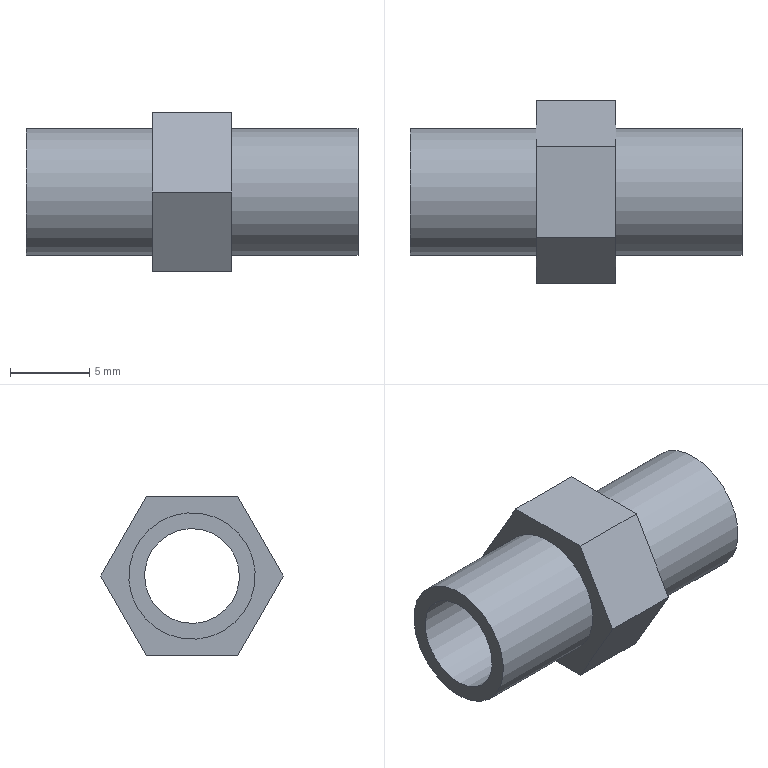Component | NX | PIPE_CAP_INTERFACE | 1 solid | 13 faces | box 21 x 11.55 x 10 mm | volume 643 mm3 | plane 10 | cylinder 3 | commonest cylinder face diameters 8 x2 6 x1
STEP:
#1=CARTESIAN_POINT('',(0.,0.,0.));
#2=DIRECTION('',(0.,0.,1.));
#3=DIRECTION('',(1.,0.,0.));
#4=AXIS2_PLACEMENT_3D('',#1,#2,#3);
#5=CARTESIAN_POINT('',(104.,-9.25,43.598));
#6=VERTEX_POINT('',#5);
#7=CARTESIAN_POINT('',(104.,-12.25,38.402));
#8=VERTEX_POINT('',#7);
#9=CARTESIAN_POINT('',(104.,-10.75,41.));
#10=DIRECTION('',(-1.,0.,0.));
#11=DIRECTION('',(0.,0.5,0.866));
#12=AXIS2_PLACEMENT_3D('',#9,#10,#11);
#13=CIRCLE('',#12,3.);
#14=CARTESIAN_POINT('',(104.,-10.75,41.));
#15=DIRECTION('',(-1.,0.,0.));
#16=DIRECTION('',(0.,0.5,0.866));
#17=AXIS2_PLACEMENT_3D('',#14,#15,#16);
#18=PLANE('',#17);
#19=CARTESIAN_POINT('',(0.,0.));
#20=DIRECTION('',(1.,0.));
#21=AXIS2_PLACEMENT_2D('',#19,#20);
#22=CIRCLE('',#21,3.);
#23=(GEOMETRIC_REPRESENTATION_CONTEXT(2)PARAMETRIC_REPRESENTATION_CONTEXT()REPRESENTATION_CONTEXT('',''));
#24=DEFINITIONAL_REPRESENTATION('',(#22),#23);
#25=PCURVE('',#18,#24);
#26=CARTESIAN_POINT('',(100.5,-10.75,41.));
#27=DIRECTION('',(1.,0.,0.));
#28=DIRECTION('',(0.,-0.5,-0.866));
#29=AXIS2_PLACEMENT_3D('',#26,#27,#28);
#30=CYLINDRICAL_SURFACE('',#29,3.);
#31=CARTESIAN_POINT('',(3.142,3.5));
#32=DIRECTION('',(-1.,0.));
#33=VECTOR('',#32,1.);
#34=LINE('',#31,#33);
#35=(GEOMETRIC_REPRESENTATION_CONTEXT(2)PARAMETRIC_REPRESENTATION_CONTEXT()REPRESENTATION_CONTEXT('',''));
#36=DEFINITIONAL_REPRESENTATION('',(#34),#35);
#37=PCURVE('',#30,#36);
#38=SURFACE_CURVE('',#13,(#25,#37),.PCURVE_S1.);
#39=EDGE_CURVE('',#6,#8,#38,.T.);
#40=ORIENTED_EDGE('',*,*,#39,.F.);
#41=CARTESIAN_POINT('',(104.,-10.75,41.));
#42=DIRECTION('',(-1.,0.,0.));
#43=DIRECTION('',(0.,0.5,0.866));
#44=AXIS2_PLACEMENT_3D('',#41,#42,#43);
#45=CIRCLE('',#44,3.);
#46=CARTESIAN_POINT('',(0.,0.));
#47=DIRECTION('',(1.,0.));
#48=AXIS2_PLACEMENT_2D('',#46,#47);
#49=CIRCLE('',#48,3.);
#50=(GEOMETRIC_REPRESENTATION_CONTEXT(2)PARAMETRIC_REPRESENTATION_CONTEXT()REPRESENTATION_CONTEXT('',''));
#51=DEFINITIONAL_REPRESENTATION('',(#49),#50);
#52=PCURVE('',#18,#51);
#53=CARTESIAN_POINT('',(9.425,3.5));
#54=DIRECTION('',(-1.,0.));
#55=VECTOR('',#54,1.);
#56=LINE('',#53,#55);
#57=(GEOMETRIC_REPRESENTATION_CONTEXT(2)PARAMETRIC_REPRESENTATION_CONTEXT()REPRESENTATION_CONTEXT('',''));
#58=DEFINITIONAL_REPRESENTATION('',(#56),#57);
#59=PCURVE('',#30,#58);
#60=SURFACE_CURVE('',#45,(#52,#59),.PCURVE_S1.);
#61=EDGE_CURVE('',#8,#6,#60,.T.);
#62=ORIENTED_EDGE('',*,*,#61,.F.);
#63=EDGE_LOOP('',(#40,#62));
#64=FACE_BOUND('',#63,.T.);
#65=CARTESIAN_POINT('',(104.,-12.75,37.536));
#66=VERTEX_POINT('',#65);
#67=CARTESIAN_POINT('',(104.,-10.75,41.));
#68=DIRECTION('',(1.,0.,0.));
#69=DIRECTION('',(0.,-0.5,-0.866));
#70=AXIS2_PLACEMENT_3D('',#67,#68,#69);
#71=CIRCLE('',#70,4.);
#72=CARTESIAN_POINT('',(-4.,0.));
#73=CARTESIAN_POINT('',(-4.,6.928));
#74=CARTESIAN_POINT('',(2.,3.464));
#75=CARTESIAN_POINT('',(8.,0.));
#76=CARTESIAN_POINT('',(2.,-3.464));
#77=CARTESIAN_POINT('',(-4.,-6.928));
#78=CARTESIAN_POINT('',(-4.,0.));
#79=(BOUNDED_CURVE()B_SPLINE_CURVE(2,(#72,#73,#74,#75,#76,#77,#78),.UNSPECIFIED.,.T.,.F.)B_SPLINE_CURVE_WITH_KNOTS((1,2,2,2,2,1),(-2.094,0.,2.094,4.189,6.283,8.378),.UNSPECIFIED.)CURVE()GEOMETRIC_REPRESENTATION_ITEM()RATIONAL_B_SPLINE_CURVE((1.,0.5,1.,0.5,1.,0.5,1.))REPRESENTATION_ITEM(''));
#80=(GEOMETRIC_REPRESENTATION_CONTEXT(2)PARAMETRIC_REPRESENTATION_CONTEXT()REPRESENTATION_CONTEXT('',''));
#81=DEFINITIONAL_REPRESENTATION('',(#79),#80);
#82=PCURVE('',#18,#81);
#83=CARTESIAN_POINT('',(104.,-10.75,41.));
#84=DIRECTION('',(1.,0.,0.));
#85=DIRECTION('',(0.,-0.5,-0.866));
#86=AXIS2_PLACEMENT_3D('',#83,#84,#85);
#87=CYLINDRICAL_SURFACE('',#86,4.);
#88=CARTESIAN_POINT('',(0.,0.));
#89=DIRECTION('',(1.,0.));
#90=VECTOR('',#89,1.);
#91=LINE('',#88,#90);
#92=(GEOMETRIC_REPRESENTATION_CONTEXT(2)PARAMETRIC_REPRESENTATION_CONTEXT()REPRESENTATION_CONTEXT('',''));
#93=DEFINITIONAL_REPRESENTATION('',(#91),#92);
#94=PCURVE('',#87,#93);
#95=SURFACE_CURVE('',#71,(#82,#94),.PCURVE_S1.);
#96=EDGE_CURVE('',#66,#66,#95,.T.);
#97=ORIENTED_EDGE('',*,*,#96,.F.);
#98=EDGE_LOOP('',(#97));
#99=FACE_BOUND('',#98,.T.);
#100=ADVANCED_FACE('',(#64,#99),#18,.T.);
#101=CARTESIAN_POINT('',(112.,-12.75,37.536));
#102=VERTEX_POINT('',#101);
#103=CARTESIAN_POINT('',(112.,-10.75,41.));
#104=DIRECTION('',(-1.,0.,0.));
#105=DIRECTION('',(0.,-0.5,-0.866));
#106=AXIS2_PLACEMENT_3D('',#103,#104,#105);
#107=CIRCLE('',#106,4.);
#108=CARTESIAN_POINT('',(6.283,8.));
#109=DIRECTION('',(-1.,0.));
#110=VECTOR('',#109,1.);
#111=LINE('',#108,#110);
#112=(GEOMETRIC_REPRESENTATION_CONTEXT(2)PARAMETRIC_REPRESENTATION_CONTEXT()REPRESENTATION_CONTEXT('',''));
#113=DEFINITIONAL_REPRESENTATION('',(#111),#112);
#114=PCURVE('',#87,#113);
#115=CARTESIAN_POINT('',(112.,-10.75,41.));
#116=DIRECTION('',(1.,0.,0.));
#117=DIRECTION('',(0.,-0.5,-0.866));
#118=AXIS2_PLACEMENT_3D('',#115,#116,#117);
#119=PLANE('',#118);
#120=CARTESIAN_POINT('',(4.,0.));
#121=CARTESIAN_POINT('',(4.,-6.928));
#122=CARTESIAN_POINT('',(-2.,-3.464));
#123=CARTESIAN_POINT('',(-8.,-0.));
#124=CARTESIAN_POINT('',(-2.,3.464));
#125=CARTESIAN_POINT('',(4.,6.928));
#126=CARTESIAN_POINT('',(4.,0.));
#127=(BOUNDED_CURVE()B_SPLINE_CURVE(2,(#120,#121,#122,#123,#124,#125,#126),.UNSPECIFIED.,.T.,.F.)B_SPLINE_CURVE_WITH_KNOTS((1,2,2,2,2,1),(-2.094,0.,2.094,4.189,6.283,8.378),.UNSPECIFIED.)CURVE()GEOMETRIC_REPRESENTATION_ITEM()RATIONAL_B_SPLINE_CURVE((1.,0.5,1.,0.5,1.,0.5,1.))REPRESENTATION_ITEM(''));
#128=(GEOMETRIC_REPRESENTATION_CONTEXT(2)PARAMETRIC_REPRESENTATION_CONTEXT()REPRESENTATION_CONTEXT('',''));
#129=DEFINITIONAL_REPRESENTATION('',(#127),#128);
#130=PCURVE('',#119,#129);
#131=SURFACE_CURVE('',#107,(#114,#130),.PCURVE_S1.);
#132=EDGE_CURVE('',#102,#102,#131,.T.);
#133=ORIENTED_EDGE('',*,*,#132,.T.);
#134=CARTESIAN_POINT('',(104.,-12.75,37.536));
#135=CARTESIAN_POINT('',(112.,-12.75,37.536));
#136=B_SPLINE_CURVE_WITH_KNOTS('',1,(#134,#135),.UNSPECIFIED.,.F.,.F.,(2,2),(0.,8.),.PIECEWISE_BEZIER_KNOTS.);
#137=CARTESIAN_POINT('',(0.,0.));
#138=DIRECTION('',(0.,1.));
#139=VECTOR('',#138,1.);
#140=LINE('',#137,#139);
#141=(GEOMETRIC_REPRESENTATION_CONTEXT(2)PARAMETRIC_REPRESENTATION_CONTEXT()REPRESENTATION_CONTEXT('',''));
#142=DEFINITIONAL_REPRESENTATION('',(#140),#141);
#143=PCURVE('',#87,#142);
#144=CARTESIAN_POINT('',(6.283,0.));
#145=DIRECTION('',(0.,1.));
#146=VECTOR('',#145,1.);
#147=LINE('',#144,#146);
#148=(GEOMETRIC_REPRESENTATION_CONTEXT(2)PARAMETRIC_REPRESENTATION_CONTEXT()REPRESENTATION_CONTEXT('',''));
#149=DEFINITIONAL_REPRESENTATION('',(#147),#148);
#150=PCURVE('',#87,#149);
#151=SEAM_CURVE('',#136,(#143,#150),.PCURVE_S1.);
#152=EDGE_CURVE('',#66,#102,#151,.T.);
#153=ORIENTED_EDGE('',*,*,#152,.F.);
#154=ORIENTED_EDGE('',*,*,#96,.T.);
#155=ORIENTED_EDGE('',*,*,#152,.T.);
#156=EDGE_LOOP('',(#133,#153,#154,#155));
#157=FACE_BOUND('',#156,.T.);
#158=ADVANCED_FACE('',(#157),#87,.T.);
#159=CARTESIAN_POINT('',(112.,-7.863,36.));
#160=VERTEX_POINT('',#159);
#161=CARTESIAN_POINT('',(112.,-4.976,41.));
#162=VERTEX_POINT('',#161);
#163=CARTESIAN_POINT('',(112.,-7.863,36.));
#164=DIRECTION('',(0.,0.5,0.866));
#165=VECTOR('',#164,1.);
#166=LINE('',#163,#165);
#167=CARTESIAN_POINT('',(117.,-7.863,36.));
#168=DIRECTION('',(0.,-0.866,0.5));
#169=DIRECTION('',(0.,-0.5,-0.866));
#170=AXIS2_PLACEMENT_3D('',#167,#168,#169);
#171=PLANE('',#170);
#172=CARTESIAN_POINT('',(0.,-5.));
#173=DIRECTION('',(-1.,0.));
#174=VECTOR('',#173,1.);
#175=LINE('',#172,#174);
#176=(GEOMETRIC_REPRESENTATION_CONTEXT(2)PARAMETRIC_REPRESENTATION_CONTEXT()REPRESENTATION_CONTEXT('',''));
#177=DEFINITIONAL_REPRESENTATION('',(#175),#176);
#178=PCURVE('',#171,#177);
#179=CARTESIAN_POINT('',(2.887,5.));
#180=DIRECTION('',(-1.,0.));
#181=VECTOR('',#180,1.);
#182=LINE('',#179,#181);
#183=(GEOMETRIC_REPRESENTATION_CONTEXT(2)PARAMETRIC_REPRESENTATION_CONTEXT()REPRESENTATION_CONTEXT('',''));
#184=DEFINITIONAL_REPRESENTATION('',(#182),#183);
#185=PCURVE('',#119,#184);
#186=SURFACE_CURVE('',#166,(#178,#185),.PCURVE_S1.);
#187=EDGE_CURVE('',#160,#162,#186,.T.);
#188=ORIENTED_EDGE('',*,*,#187,.T.);
#189=CARTESIAN_POINT('',(117.,-4.976,41.));
#190=VERTEX_POINT('',#189);
#191=CARTESIAN_POINT('',(117.,-4.976,41.));
#192=DIRECTION('',(-1.,0.,0.));
#193=VECTOR('',#192,1.);
#194=LINE('',#191,#193);
#195=CARTESIAN_POINT('',(-5.774,0.));
#196=DIRECTION('',(0.,-1.));
#197=VECTOR('',#196,1.);
#198=LINE('',#195,#197);
#199=(GEOMETRIC_REPRESENTATION_CONTEXT(2)PARAMETRIC_REPRESENTATION_CONTEXT()REPRESENTATION_CONTEXT('',''));
#200=DEFINITIONAL_REPRESENTATION('',(#198),#199);
#201=PCURVE('',#171,#200);
#202=CARTESIAN_POINT('',(117.,-4.976,41.));
#203=DIRECTION('',(0.,-0.866,-0.5));
#204=DIRECTION('',(0.,0.5,-0.866));
#205=AXIS2_PLACEMENT_3D('',#202,#203,#204);
#206=PLANE('',#205);
#207=CARTESIAN_POINT('',(0.,0.));
#208=DIRECTION('',(0.,-1.));
#209=VECTOR('',#208,1.);
#210=LINE('',#207,#209);
#211=(GEOMETRIC_REPRESENTATION_CONTEXT(2)PARAMETRIC_REPRESENTATION_CONTEXT()REPRESENTATION_CONTEXT('',''));
#212=DEFINITIONAL_REPRESENTATION('',(#210),#211);
#213=PCURVE('',#206,#212);
#214=SURFACE_CURVE('',#194,(#201,#213),.PCURVE_S1.);
#215=EDGE_CURVE('',#190,#162,#214,.T.);
#216=ORIENTED_EDGE('',*,*,#215,.F.);
#217=CARTESIAN_POINT('',(117.,-7.863,36.));
#218=VERTEX_POINT('',#217);
#219=CARTESIAN_POINT('',(117.,-7.863,36.));
#220=DIRECTION('',(0.,0.5,0.866));
#221=VECTOR('',#220,1.);
#222=LINE('',#219,#221);
#223=CARTESIAN_POINT('',(0.,0.));
#224=DIRECTION('',(-1.,0.));
#225=VECTOR('',#224,1.);
#226=LINE('',#223,#225);
#227=(GEOMETRIC_REPRESENTATION_CONTEXT(2)PARAMETRIC_REPRESENTATION_CONTEXT()REPRESENTATION_CONTEXT('',''));
#228=DEFINITIONAL_REPRESENTATION('',(#226),#227);
#229=PCURVE('',#171,#228);
#230=CARTESIAN_POINT('',(117.,-10.75,41.));
#231=DIRECTION('',(1.,0.,0.));
#232=DIRECTION('',(0.,-0.5,-0.866));
#233=AXIS2_PLACEMENT_3D('',#230,#231,#232);
#234=PLANE('',#233);
#235=CARTESIAN_POINT('',(2.887,5.));
#236=DIRECTION('',(-1.,0.));
#237=VECTOR('',#236,1.);
#238=LINE('',#235,#237);
#239=(GEOMETRIC_REPRESENTATION_CONTEXT(2)PARAMETRIC_REPRESENTATION_CONTEXT()REPRESENTATION_CONTEXT('',''));
#240=DEFINITIONAL_REPRESENTATION('',(#238),#239);
#241=PCURVE('',#234,#240);
#242=SURFACE_CURVE('',#222,(#229,#241),.PCURVE_S1.);
#243=EDGE_CURVE('',#218,#190,#242,.T.);
#244=ORIENTED_EDGE('',*,*,#243,.F.);
#245=CARTESIAN_POINT('',(117.,-7.863,36.));
#246=DIRECTION('',(-1.,0.,0.));
#247=VECTOR('',#246,1.);
#248=LINE('',#245,#247);
#249=CARTESIAN_POINT('',(0.,0.));
#250=DIRECTION('',(0.,-1.));
#251=VECTOR('',#250,1.);
#252=LINE('',#249,#251);
#253=(GEOMETRIC_REPRESENTATION_CONTEXT(2)PARAMETRIC_REPRESENTATION_CONTEXT()REPRESENTATION_CONTEXT('',''));
#254=DEFINITIONAL_REPRESENTATION('',(#252),#253);
#255=PCURVE('',#171,#254);
#256=CARTESIAN_POINT('',(117.,-13.637,36.));
#257=DIRECTION('',(0.,0.,1.));
#258=DIRECTION('',(0.,-1.,0.));
#259=AXIS2_PLACEMENT_3D('',#256,#257,#258);
#260=PLANE('',#259);
#261=CARTESIAN_POINT('',(-5.774,0.));
#262=DIRECTION('',(0.,-1.));
#263=VECTOR('',#262,1.);
#264=LINE('',#261,#263);
#265=(GEOMETRIC_REPRESENTATION_CONTEXT(2)PARAMETRIC_REPRESENTATION_CONTEXT()REPRESENTATION_CONTEXT('',''));
#266=DEFINITIONAL_REPRESENTATION('',(#264),#265);
#267=PCURVE('',#260,#266);
#268=SURFACE_CURVE('',#248,(#255,#267),.PCURVE_S1.);
#269=EDGE_CURVE('',#218,#160,#268,.T.);
#270=ORIENTED_EDGE('',*,*,#269,.T.);
#271=EDGE_LOOP('',(#188,#216,#244,#270));
#272=FACE_BOUND('',#271,.T.);
#273=ADVANCED_FACE('',(#272),#171,.F.);
#274=CARTESIAN_POINT('',(112.,-7.863,46.));
#275=VERTEX_POINT('',#274);
#276=CARTESIAN_POINT('',(112.,-4.976,41.));
#277=DIRECTION('',(0.,-0.5,0.866));
#278=VECTOR('',#277,1.);
#279=LINE('',#276,#278);
#280=CARTESIAN_POINT('',(0.,-5.));
#281=DIRECTION('',(-1.,0.));
#282=VECTOR('',#281,1.);
#283=LINE('',#280,#282);
#284=(GEOMETRIC_REPRESENTATION_CONTEXT(2)PARAMETRIC_REPRESENTATION_CONTEXT()REPRESENTATION_CONTEXT('',''));
#285=DEFINITIONAL_REPRESENTATION('',(#283),#284);
#286=PCURVE('',#206,#285);
#287=CARTESIAN_POINT('',(-2.887,5.));
#288=DIRECTION('',(-0.5,-0.866));
#289=VECTOR('',#288,1.);
#290=LINE('',#287,#289);
#291=(GEOMETRIC_REPRESENTATION_CONTEXT(2)PARAMETRIC_REPRESENTATION_CONTEXT()REPRESENTATION_CONTEXT('',''));
#292=DEFINITIONAL_REPRESENTATION('',(#290),#291);
#293=PCURVE('',#119,#292);
#294=SURFACE_CURVE('',#279,(#286,#293),.PCURVE_S1.);
#295=EDGE_CURVE('',#162,#275,#294,.T.);
#296=ORIENTED_EDGE('',*,*,#295,.T.);
#297=CARTESIAN_POINT('',(117.,-7.863,46.));
#298=VERTEX_POINT('',#297);
#299=CARTESIAN_POINT('',(117.,-7.863,46.));
#300=DIRECTION('',(-1.,0.,0.));
#301=VECTOR('',#300,1.);
#302=LINE('',#299,#301);
#303=CARTESIAN_POINT('',(-5.774,0.));
#304=DIRECTION('',(0.,-1.));
#305=VECTOR('',#304,1.);
#306=LINE('',#303,#305);
#307=(GEOMETRIC_REPRESENTATION_CONTEXT(2)PARAMETRIC_REPRESENTATION_CONTEXT()REPRESENTATION_CONTEXT('',''));
#308=DEFINITIONAL_REPRESENTATION('',(#306),#307);
#309=PCURVE('',#206,#308);
#310=CARTESIAN_POINT('',(117.,-7.863,46.));
#311=DIRECTION('',(0.,-0.,-1.));
#312=DIRECTION('',(0.,1.,-0.));
#313=AXIS2_PLACEMENT_3D('',#310,#311,#312);
#314=PLANE('',#313);
#315=CARTESIAN_POINT('',(0.,0.));
#316=DIRECTION('',(0.,-1.));
#317=VECTOR('',#316,1.);
#318=LINE('',#315,#317);
#319=(GEOMETRIC_REPRESENTATION_CONTEXT(2)PARAMETRIC_REPRESENTATION_CONTEXT()REPRESENTATION_CONTEXT('',''));
#320=DEFINITIONAL_REPRESENTATION('',(#318),#319);
#321=PCURVE('',#314,#320);
#322=SURFACE_CURVE('',#302,(#309,#321),.PCURVE_S1.);
#323=EDGE_CURVE('',#298,#275,#322,.T.);
#324=ORIENTED_EDGE('',*,*,#323,.F.);
#325=CARTESIAN_POINT('',(117.,-4.976,41.));
#326=DIRECTION('',(0.,-0.5,0.866));
#327=VECTOR('',#326,1.);
#328=LINE('',#325,#327);
#329=CARTESIAN_POINT('',(0.,0.));
#330=DIRECTION('',(-1.,0.));
#331=VECTOR('',#330,1.);
#332=LINE('',#329,#331);
#333=(GEOMETRIC_REPRESENTATION_CONTEXT(2)PARAMETRIC_REPRESENTATION_CONTEXT()REPRESENTATION_CONTEXT('',''));
#334=DEFINITIONAL_REPRESENTATION('',(#332),#333);
#335=PCURVE('',#206,#334);
#336=CARTESIAN_POINT('',(-2.887,5.));
#337=DIRECTION('',(-0.5,-0.866));
#338=VECTOR('',#337,1.);
#339=LINE('',#336,#338);
#340=(GEOMETRIC_REPRESENTATION_CONTEXT(2)PARAMETRIC_REPRESENTATION_CONTEXT()REPRESENTATION_CONTEXT('',''));
#341=DEFINITIONAL_REPRESENTATION('',(#339),#340);
#342=PCURVE('',#234,#341);
#343=SURFACE_CURVE('',#328,(#335,#342),.PCURVE_S1.);
#344=EDGE_CURVE('',#190,#298,#343,.T.);
#345=ORIENTED_EDGE('',*,*,#344,.F.);
#346=ORIENTED_EDGE('',*,*,#215,.T.);
#347=EDGE_LOOP('',(#296,#324,#345,#346));
#348=FACE_BOUND('',#347,.T.);
#349=ADVANCED_FACE('',(#348),#206,.F.);
#350=CARTESIAN_POINT('',(112.,-13.637,46.));
#351=VERTEX_POINT('',#350);
#352=CARTESIAN_POINT('',(112.,-7.863,46.));
#353=DIRECTION('',(0.,-1.,0.));
#354=VECTOR('',#353,1.);
#355=LINE('',#352,#354);
#356=CARTESIAN_POINT('',(0.,-5.));
#357=DIRECTION('',(-1.,0.));
#358=VECTOR('',#357,1.);
#359=LINE('',#356,#358);
#360=(GEOMETRIC_REPRESENTATION_CONTEXT(2)PARAMETRIC_REPRESENTATION_CONTEXT()REPRESENTATION_CONTEXT('',''));
#361=DEFINITIONAL_REPRESENTATION('',(#359),#360);
#362=PCURVE('',#314,#361);
#363=CARTESIAN_POINT('',(-5.774,-0.));
#364=DIRECTION('',(0.5,-0.866));
#365=VECTOR('',#364,1.);
#366=LINE('',#363,#365);
#367=(GEOMETRIC_REPRESENTATION_CONTEXT(2)PARAMETRIC_REPRESENTATION_CONTEXT()REPRESENTATION_CONTEXT('',''));
#368=DEFINITIONAL_REPRESENTATION('',(#366),#367);
#369=PCURVE('',#119,#368);
#370=SURFACE_CURVE('',#355,(#362,#369),.PCURVE_S1.);
#371=EDGE_CURVE('',#275,#351,#370,.T.);
#372=ORIENTED_EDGE('',*,*,#371,.T.);
#373=CARTESIAN_POINT('',(117.,-13.637,46.));
#374=VERTEX_POINT('',#373);
#375=CARTESIAN_POINT('',(117.,-13.637,46.));
#376=DIRECTION('',(-1.,0.,0.));
#377=VECTOR('',#376,1.);
#378=LINE('',#375,#377);
#379=CARTESIAN_POINT('',(-5.774,0.));
#380=DIRECTION('',(0.,-1.));
#381=VECTOR('',#380,1.);
#382=LINE('',#379,#381);
#383=(GEOMETRIC_REPRESENTATION_CONTEXT(2)PARAMETRIC_REPRESENTATION_CONTEXT()REPRESENTATION_CONTEXT('',''));
#384=DEFINITIONAL_REPRESENTATION('',(#382),#383);
#385=PCURVE('',#314,#384);
#386=CARTESIAN_POINT('',(117.,-13.637,46.));
#387=DIRECTION('',(0.,0.866,-0.5));
#388=DIRECTION('',(0.,0.5,0.866));
#389=AXIS2_PLACEMENT_3D('',#386,#387,#388);
#390=PLANE('',#389);
#391=CARTESIAN_POINT('',(0.,0.));
#392=DIRECTION('',(0.,-1.));
#393=VECTOR('',#392,1.);
#394=LINE('',#391,#393);
#395=(GEOMETRIC_REPRESENTATION_CONTEXT(2)PARAMETRIC_REPRESENTATION_CONTEXT()REPRESENTATION_CONTEXT('',''));
#396=DEFINITIONAL_REPRESENTATION('',(#394),#395);
#397=PCURVE('',#390,#396);
#398=SURFACE_CURVE('',#378,(#385,#397),.PCURVE_S1.);
#399=EDGE_CURVE('',#374,#351,#398,.T.);
#400=ORIENTED_EDGE('',*,*,#399,.F.);
#401=CARTESIAN_POINT('',(117.,-7.863,46.));
#402=DIRECTION('',(0.,-1.,0.));
#403=VECTOR('',#402,1.);
#404=LINE('',#401,#403);
#405=CARTESIAN_POINT('',(0.,0.));
#406=DIRECTION('',(-1.,0.));
#407=VECTOR('',#406,1.);
#408=LINE('',#405,#407);
#409=(GEOMETRIC_REPRESENTATION_CONTEXT(2)PARAMETRIC_REPRESENTATION_CONTEXT()REPRESENTATION_CONTEXT('',''));
#410=DEFINITIONAL_REPRESENTATION('',(#408),#409);
#411=PCURVE('',#314,#410);
#412=CARTESIAN_POINT('',(-5.774,-0.));
#413=DIRECTION('',(0.5,-0.866));
#414=VECTOR('',#413,1.);
#415=LINE('',#412,#414);
#416=(GEOMETRIC_REPRESENTATION_CONTEXT(2)PARAMETRIC_REPRESENTATION_CONTEXT()REPRESENTATION_CONTEXT('',''));
#417=DEFINITIONAL_REPRESENTATION('',(#415),#416);
#418=PCURVE('',#234,#417);
#419=SURFACE_CURVE('',#404,(#411,#418),.PCURVE_S1.);
#420=EDGE_CURVE('',#298,#374,#419,.T.);
#421=ORIENTED_EDGE('',*,*,#420,.F.);
#422=ORIENTED_EDGE('',*,*,#323,.T.);
#423=EDGE_LOOP('',(#372,#400,#421,#422));
#424=FACE_BOUND('',#423,.T.);
#425=ADVANCED_FACE('',(#424),#314,.F.);
#426=CARTESIAN_POINT('',(112.,-16.524,41.));
#427=VERTEX_POINT('',#426);
#428=CARTESIAN_POINT('',(112.,-13.637,46.));
#429=DIRECTION('',(0.,-0.5,-0.866));
#430=VECTOR('',#429,1.);
#431=LINE('',#428,#430);
#432=CARTESIAN_POINT('',(0.,-5.));
#433=DIRECTION('',(-1.,0.));
#434=VECTOR('',#433,1.);
#435=LINE('',#432,#434);
#436=(GEOMETRIC_REPRESENTATION_CONTEXT(2)PARAMETRIC_REPRESENTATION_CONTEXT()REPRESENTATION_CONTEXT('',''));
#437=DEFINITIONAL_REPRESENTATION('',(#435),#436);
#438=PCURVE('',#390,#437);
#439=CARTESIAN_POINT('',(-2.887,-5.));
#440=DIRECTION('',(1.,-0.));
#441=VECTOR('',#440,1.);
#442=LINE('',#439,#441);
#443=(GEOMETRIC_REPRESENTATION_CONTEXT(2)PARAMETRIC_REPRESENTATION_CONTEXT()REPRESENTATION_CONTEXT('',''));
#444=DEFINITIONAL_REPRESENTATION('',(#442),#443);
#445=PCURVE('',#119,#444);
#446=SURFACE_CURVE('',#431,(#438,#445),.PCURVE_S1.);
#447=EDGE_CURVE('',#351,#427,#446,.T.);
#448=ORIENTED_EDGE('',*,*,#447,.T.);
#449=CARTESIAN_POINT('',(117.,-16.524,41.));
#450=VERTEX_POINT('',#449);
#451=CARTESIAN_POINT('',(117.,-16.524,41.));
#452=DIRECTION('',(-1.,0.,0.));
#453=VECTOR('',#452,1.);
#454=LINE('',#451,#453);
#455=CARTESIAN_POINT('',(-5.774,0.));
#456=DIRECTION('',(0.,-1.));
#457=VECTOR('',#456,1.);
#458=LINE('',#455,#457);
#459=(GEOMETRIC_REPRESENTATION_CONTEXT(2)PARAMETRIC_REPRESENTATION_CONTEXT()REPRESENTATION_CONTEXT('',''));
#460=DEFINITIONAL_REPRESENTATION('',(#458),#459);
#461=PCURVE('',#390,#460);
#462=CARTESIAN_POINT('',(117.,-16.524,41.));
#463=DIRECTION('',(0.,0.866,0.5));
#464=DIRECTION('',(0.,-0.5,0.866));
#465=AXIS2_PLACEMENT_3D('',#462,#463,#464);
#466=PLANE('',#465);
#467=CARTESIAN_POINT('',(0.,0.));
#468=DIRECTION('',(0.,-1.));
#469=VECTOR('',#468,1.);
#470=LINE('',#467,#469);
#471=(GEOMETRIC_REPRESENTATION_CONTEXT(2)PARAMETRIC_REPRESENTATION_CONTEXT()REPRESENTATION_CONTEXT('',''));
#472=DEFINITIONAL_REPRESENTATION('',(#470),#471);
#473=PCURVE('',#466,#472);
#474=SURFACE_CURVE('',#454,(#461,#473),.PCURVE_S1.);
#475=EDGE_CURVE('',#450,#427,#474,.T.);
#476=ORIENTED_EDGE('',*,*,#475,.F.);
#477=CARTESIAN_POINT('',(117.,-13.637,46.));
#478=DIRECTION('',(0.,-0.5,-0.866));
#479=VECTOR('',#478,1.);
#480=LINE('',#477,#479);
#481=CARTESIAN_POINT('',(0.,0.));
#482=DIRECTION('',(-1.,0.));
#483=VECTOR('',#482,1.);
#484=LINE('',#481,#483);
#485=(GEOMETRIC_REPRESENTATION_CONTEXT(2)PARAMETRIC_REPRESENTATION_CONTEXT()REPRESENTATION_CONTEXT('',''));
#486=DEFINITIONAL_REPRESENTATION('',(#484),#485);
#487=PCURVE('',#390,#486);
#488=CARTESIAN_POINT('',(-2.887,-5.));
#489=DIRECTION('',(1.,-0.));
#490=VECTOR('',#489,1.);
#491=LINE('',#488,#490);
#492=(GEOMETRIC_REPRESENTATION_CONTEXT(2)PARAMETRIC_REPRESENTATION_CONTEXT()REPRESENTATION_CONTEXT('',''));
#493=DEFINITIONAL_REPRESENTATION('',(#491),#492);
#494=PCURVE('',#234,#493);
#495=SURFACE_CURVE('',#480,(#487,#494),.PCURVE_S1.);
#496=EDGE_CURVE('',#374,#450,#495,.T.);
#497=ORIENTED_EDGE('',*,*,#496,.F.);
#498=ORIENTED_EDGE('',*,*,#399,.T.);
#499=EDGE_LOOP('',(#448,#476,#497,#498));
#500=FACE_BOUND('',#499,.T.);
#501=ADVANCED_FACE('',(#500),#390,.F.);
#502=CARTESIAN_POINT('',(112.,-13.637,36.));
#503=VERTEX_POINT('',#502);
#504=CARTESIAN_POINT('',(112.,-16.524,41.));
#505=DIRECTION('',(0.,0.5,-0.866));
#506=VECTOR('',#505,1.);
#507=LINE('',#504,#506);
#508=CARTESIAN_POINT('',(0.,-5.));
#509=DIRECTION('',(-1.,0.));
#510=VECTOR('',#509,1.);
#511=LINE('',#508,#510);
#512=(GEOMETRIC_REPRESENTATION_CONTEXT(2)PARAMETRIC_REPRESENTATION_CONTEXT()REPRESENTATION_CONTEXT('',''));
#513=DEFINITIONAL_REPRESENTATION('',(#511),#512);
#514=PCURVE('',#466,#513);
#515=CARTESIAN_POINT('',(2.887,-5.));
#516=DIRECTION('',(0.5,0.866));
#517=VECTOR('',#516,1.);
#518=LINE('',#515,#517);
#519=(GEOMETRIC_REPRESENTATION_CONTEXT(2)PARAMETRIC_REPRESENTATION_CONTEXT()REPRESENTATION_CONTEXT('',''));
#520=DEFINITIONAL_REPRESENTATION('',(#518),#519);
#521=PCURVE('',#119,#520);
#522=SURFACE_CURVE('',#507,(#514,#521),.PCURVE_S1.);
#523=EDGE_CURVE('',#427,#503,#522,.T.);
#524=ORIENTED_EDGE('',*,*,#523,.T.);
#525=CARTESIAN_POINT('',(117.,-13.637,36.));
#526=VERTEX_POINT('',#525);
#527=CARTESIAN_POINT('',(117.,-13.637,36.));
#528=DIRECTION('',(-1.,0.,0.));
#529=VECTOR('',#528,1.);
#530=LINE('',#527,#529);
#531=CARTESIAN_POINT('',(-5.774,0.));
#532=DIRECTION('',(0.,-1.));
#533=VECTOR('',#532,1.);
#534=LINE('',#531,#533);
#535=(GEOMETRIC_REPRESENTATION_CONTEXT(2)PARAMETRIC_REPRESENTATION_CONTEXT()REPRESENTATION_CONTEXT('',''));
#536=DEFINITIONAL_REPRESENTATION('',(#534),#535);
#537=PCURVE('',#466,#536);
#538=CARTESIAN_POINT('',(0.,0.));
#539=DIRECTION('',(0.,-1.));
#540=VECTOR('',#539,1.);
#541=LINE('',#538,#540);
#542=(GEOMETRIC_REPRESENTATION_CONTEXT(2)PARAMETRIC_REPRESENTATION_CONTEXT()REPRESENTATION_CONTEXT('',''));
#543=DEFINITIONAL_REPRESENTATION('',(#541),#542);
#544=PCURVE('',#260,#543);
#545=SURFACE_CURVE('',#530,(#537,#544),.PCURVE_S1.);
#546=EDGE_CURVE('',#526,#503,#545,.T.);
#547=ORIENTED_EDGE('',*,*,#546,.F.);
#548=CARTESIAN_POINT('',(117.,-16.524,41.));
#549=DIRECTION('',(0.,0.5,-0.866));
#550=VECTOR('',#549,1.);
#551=LINE('',#548,#550);
#552=CARTESIAN_POINT('',(0.,0.));
#553=DIRECTION('',(-1.,0.));
#554=VECTOR('',#553,1.);
#555=LINE('',#552,#554);
#556=(GEOMETRIC_REPRESENTATION_CONTEXT(2)PARAMETRIC_REPRESENTATION_CONTEXT()REPRESENTATION_CONTEXT('',''));
#557=DEFINITIONAL_REPRESENTATION('',(#555),#556);
#558=PCURVE('',#466,#557);
#559=CARTESIAN_POINT('',(2.887,-5.));
#560=DIRECTION('',(0.5,0.866));
#561=VECTOR('',#560,1.);
#562=LINE('',#559,#561);
#563=(GEOMETRIC_REPRESENTATION_CONTEXT(2)PARAMETRIC_REPRESENTATION_CONTEXT()REPRESENTATION_CONTEXT('',''));
#564=DEFINITIONAL_REPRESENTATION('',(#562),#563);
#565=PCURVE('',#234,#564);
#566=SURFACE_CURVE('',#551,(#558,#565),.PCURVE_S1.);
#567=EDGE_CURVE('',#450,#526,#566,.T.);
#568=ORIENTED_EDGE('',*,*,#567,.F.);
#569=ORIENTED_EDGE('',*,*,#475,.T.);
#570=EDGE_LOOP('',(#524,#547,#568,#569));
#571=FACE_BOUND('',#570,.T.);
#572=ADVANCED_FACE('',(#571),#466,.F.);
#573=CARTESIAN_POINT('',(112.,-13.637,36.));
#574=DIRECTION('',(0.,1.,-0.));
#575=VECTOR('',#574,1.);
#576=LINE('',#573,#575);
#577=CARTESIAN_POINT('',(0.,-5.));
#578=DIRECTION('',(-1.,0.));
#579=VECTOR('',#578,1.);
#580=LINE('',#577,#579);
#581=(GEOMETRIC_REPRESENTATION_CONTEXT(2)PARAMETRIC_REPRESENTATION_CONTEXT()REPRESENTATION_CONTEXT('',''));
#582=DEFINITIONAL_REPRESENTATION('',(#580),#581);
#583=PCURVE('',#260,#582);
#584=CARTESIAN_POINT('',(5.774,0.));
#585=DIRECTION('',(-0.5,0.866));
#586=VECTOR('',#585,1.);
#587=LINE('',#584,#586);
#588=(GEOMETRIC_REPRESENTATION_CONTEXT(2)PARAMETRIC_REPRESENTATION_CONTEXT()REPRESENTATION_CONTEXT('',''));
#589=DEFINITIONAL_REPRESENTATION('',(#587),#588);
#590=PCURVE('',#119,#589);
#591=SURFACE_CURVE('',#576,(#583,#590),.PCURVE_S1.);
#592=EDGE_CURVE('',#503,#160,#591,.T.);
#593=ORIENTED_EDGE('',*,*,#592,.T.);
#594=ORIENTED_EDGE('',*,*,#269,.F.);
#595=CARTESIAN_POINT('',(117.,-13.637,36.));
#596=DIRECTION('',(0.,1.,-0.));
#597=VECTOR('',#596,1.);
#598=LINE('',#595,#597);
#599=CARTESIAN_POINT('',(0.,0.));
#600=DIRECTION('',(-1.,0.));
#601=VECTOR('',#600,1.);
#602=LINE('',#599,#601);
#603=(GEOMETRIC_REPRESENTATION_CONTEXT(2)PARAMETRIC_REPRESENTATION_CONTEXT()REPRESENTATION_CONTEXT('',''));
#604=DEFINITIONAL_REPRESENTATION('',(#602),#603);
#605=PCURVE('',#260,#604);
#606=CARTESIAN_POINT('',(5.774,0.));
#607=DIRECTION('',(-0.5,0.866));
#608=VECTOR('',#607,1.);
#609=LINE('',#606,#608);
#610=(GEOMETRIC_REPRESENTATION_CONTEXT(2)PARAMETRIC_REPRESENTATION_CONTEXT()REPRESENTATION_CONTEXT('',''));
#611=DEFINITIONAL_REPRESENTATION('',(#609),#610);
#612=PCURVE('',#234,#611);
#613=SURFACE_CURVE('',#598,(#605,#612),.PCURVE_S1.);
#614=EDGE_CURVE('',#526,#218,#613,.T.);
#615=ORIENTED_EDGE('',*,*,#614,.F.);
#616=ORIENTED_EDGE('',*,*,#546,.T.);
#617=EDGE_LOOP('',(#593,#594,#615,#616));
#618=FACE_BOUND('',#617,.T.);
#619=ADVANCED_FACE('',(#618),#260,.F.);
#620=CARTESIAN_POINT('',(117.,-8.75,37.536));
#621=VERTEX_POINT('',#620);
#622=CARTESIAN_POINT('',(117.,-10.75,41.));
#623=DIRECTION('',(-1.,0.,0.));
#624=DIRECTION('',(0.,0.5,-0.866));
#625=AXIS2_PLACEMENT_3D('',#622,#623,#624);
#626=CIRCLE('',#625,4.);
#627=CARTESIAN_POINT('',(2.,3.464));
#628=CARTESIAN_POINT('',(8.,-0.));
#629=CARTESIAN_POINT('',(2.,-3.464));
#630=CARTESIAN_POINT('',(-4.,-6.928));
#631=CARTESIAN_POINT('',(-4.,0.));
#632=CARTESIAN_POINT('',(-4.,6.928));
#633=CARTESIAN_POINT('',(2.,3.464));
#634=(BOUNDED_CURVE()B_SPLINE_CURVE(2,(#627,#628,#629,#630,#631,#632,#633),.UNSPECIFIED.,.T.,.F.)B_SPLINE_CURVE_WITH_KNOTS((1,2,2,2,2,1),(-2.094,0.,2.094,4.189,6.283,8.378),.UNSPECIFIED.)CURVE()GEOMETRIC_REPRESENTATION_ITEM()RATIONAL_B_SPLINE_CURVE((1.,0.5,1.,0.5,1.,0.5,1.))REPRESENTATION_ITEM(''));
#635=(GEOMETRIC_REPRESENTATION_CONTEXT(2)PARAMETRIC_REPRESENTATION_CONTEXT()REPRESENTATION_CONTEXT('',''));
#636=DEFINITIONAL_REPRESENTATION('',(#634),#635);
#637=PCURVE('',#234,#636);
#638=CARTESIAN_POINT('',(125.,-10.75,41.));
#639=DIRECTION('',(-1.,0.,0.));
#640=DIRECTION('',(0.,0.5,0.866));
#641=AXIS2_PLACEMENT_3D('',#638,#639,#640);
#642=CYLINDRICAL_SURFACE('',#641,4.);
#643=CARTESIAN_POINT('',(2.094,8.));
#644=DIRECTION('',(1.,0.));
#645=VECTOR('',#644,1.);
#646=LINE('',#643,#645);
#647=(GEOMETRIC_REPRESENTATION_CONTEXT(2)PARAMETRIC_REPRESENTATION_CONTEXT()REPRESENTATION_CONTEXT('',''));
#648=DEFINITIONAL_REPRESENTATION('',(#646),#647);
#649=PCURVE('',#642,#648);
#650=SURFACE_CURVE('',#626,(#637,#649),.PCURVE_S1.);
#651=EDGE_CURVE('',#621,#621,#650,.T.);
#652=ORIENTED_EDGE('',*,*,#651,.T.);
#653=EDGE_LOOP('',(#652));
#654=FACE_BOUND('',#653,.T.);
#655=ORIENTED_EDGE('',*,*,#243,.T.);
#656=ORIENTED_EDGE('',*,*,#344,.T.);
#657=ORIENTED_EDGE('',*,*,#420,.T.);
#658=ORIENTED_EDGE('',*,*,#496,.T.);
#659=ORIENTED_EDGE('',*,*,#567,.T.);
#660=ORIENTED_EDGE('',*,*,#614,.T.);
#661=EDGE_LOOP('',(#655,#656,#657,#658,#659,#660));
#662=FACE_BOUND('',#661,.T.);
#663=ADVANCED_FACE('',(#654,#662),#234,.T.);
#664=ORIENTED_EDGE('',*,*,#132,.F.);
#665=EDGE_LOOP('',(#664));
#666=FACE_BOUND('',#665,.T.);
#667=ORIENTED_EDGE('',*,*,#187,.F.);
#668=ORIENTED_EDGE('',*,*,#592,.F.);
#669=ORIENTED_EDGE('',*,*,#523,.F.);
#670=ORIENTED_EDGE('',*,*,#447,.F.);
#671=ORIENTED_EDGE('',*,*,#371,.F.);
#672=ORIENTED_EDGE('',*,*,#295,.F.);
#673=EDGE_LOOP('',(#667,#668,#669,#670,#671,#672));
#674=FACE_BOUND('',#673,.T.);
#675=ADVANCED_FACE('',(#666,#674),#119,.F.);
#676=CARTESIAN_POINT('',(125.,-8.75,37.536));
#677=VERTEX_POINT('',#676);
#678=CARTESIAN_POINT('',(125.,-10.75,41.));
#679=DIRECTION('',(-1.,0.,0.));
#680=DIRECTION('',(0.,0.5,-0.866));
#681=AXIS2_PLACEMENT_3D('',#678,#679,#680);
#682=CIRCLE('',#681,4.);
#683=CARTESIAN_POINT('',(2.094,0.));
#684=DIRECTION('',(1.,0.));
#685=VECTOR('',#684,1.);
#686=LINE('',#683,#685);
#687=(GEOMETRIC_REPRESENTATION_CONTEXT(2)PARAMETRIC_REPRESENTATION_CONTEXT()REPRESENTATION_CONTEXT('',''));
#688=DEFINITIONAL_REPRESENTATION('',(#686),#687);
#689=PCURVE('',#642,#688);
#690=CARTESIAN_POINT('',(125.,-10.75,41.));
#691=DIRECTION('',(-1.,0.,0.));
#692=DIRECTION('',(0.,0.5,0.866));
#693=AXIS2_PLACEMENT_3D('',#690,#691,#692);
#694=PLANE('',#693);
#695=CARTESIAN_POINT('',(0.,0.));
#696=DIRECTION('',(-0.5,0.866));
#697=AXIS2_PLACEMENT_2D('',#695,#696);
#698=CIRCLE('',#697,4.);
#699=(GEOMETRIC_REPRESENTATION_CONTEXT(2)PARAMETRIC_REPRESENTATION_CONTEXT()REPRESENTATION_CONTEXT('',''));
#700=DEFINITIONAL_REPRESENTATION('',(#698),#699);
#701=PCURVE('',#694,#700);
#702=SURFACE_CURVE('',#682,(#689,#701),.PCURVE_S1.);
#703=EDGE_CURVE('',#677,#677,#702,.T.);
#704=ORIENTED_EDGE('',*,*,#703,.T.);
#705=CARTESIAN_POINT('',(125.,-8.75,37.536));
#706=CARTESIAN_POINT('',(117.,-8.75,37.536));
#707=B_SPLINE_CURVE_WITH_KNOTS('',1,(#705,#706),.UNSPECIFIED.,.F.,.F.,(2,2),(0.,8.),.PIECEWISE_BEZIER_KNOTS.);
#708=CARTESIAN_POINT('',(8.378,0.));
#709=DIRECTION('',(0.,1.));
#710=VECTOR('',#709,1.);
#711=LINE('',#708,#710);
#712=(GEOMETRIC_REPRESENTATION_CONTEXT(2)PARAMETRIC_REPRESENTATION_CONTEXT()REPRESENTATION_CONTEXT('',''));
#713=DEFINITIONAL_REPRESENTATION('',(#711),#712);
#714=PCURVE('',#642,#713);
#715=CARTESIAN_POINT('',(2.094,0.));
#716=DIRECTION('',(0.,1.));
#717=VECTOR('',#716,1.);
#718=LINE('',#715,#717);
#719=(GEOMETRIC_REPRESENTATION_CONTEXT(2)PARAMETRIC_REPRESENTATION_CONTEXT()REPRESENTATION_CONTEXT('',''));
#720=DEFINITIONAL_REPRESENTATION('',(#718),#719);
#721=PCURVE('',#642,#720);
#722=SEAM_CURVE('',#707,(#714,#721),.PCURVE_S1.);
#723=EDGE_CURVE('',#677,#621,#722,.T.);
#724=ORIENTED_EDGE('',*,*,#723,.T.);
#725=ORIENTED_EDGE('',*,*,#651,.F.);
#726=ORIENTED_EDGE('',*,*,#723,.F.);
#727=EDGE_LOOP('',(#704,#724,#725,#726));
#728=FACE_BOUND('',#727,.T.);
#729=ADVANCED_FACE('',(#728),#642,.T.);
#730=CARTESIAN_POINT('',(125.,-12.25,38.402));
#731=VERTEX_POINT('',#730);
#732=CARTESIAN_POINT('',(125.,-10.75,41.));
#733=DIRECTION('',(1.,0.,0.));
#734=DIRECTION('',(0.,-0.5,-0.866));
#735=AXIS2_PLACEMENT_3D('',#732,#733,#734);
#736=CIRCLE('',#735,3.);
#737=CARTESIAN_POINT('',(-3.,-0.));
#738=CARTESIAN_POINT('',(-3.,5.196));
#739=CARTESIAN_POINT('',(1.5,2.598));
#740=CARTESIAN_POINT('',(6.,0.));
#741=CARTESIAN_POINT('',(1.5,-2.598));
#742=CARTESIAN_POINT('',(-3.,-5.196));
#743=CARTESIAN_POINT('',(-3.,-0.));
#744=(BOUNDED_CURVE()B_SPLINE_CURVE(2,(#737,#738,#739,#740,#741,#742,#743),.UNSPECIFIED.,.T.,.F.)B_SPLINE_CURVE_WITH_KNOTS((1,2,2,2,2,1),(-2.094,0.,2.094,4.189,6.283,8.378),.UNSPECIFIED.)CURVE()GEOMETRIC_REPRESENTATION_ITEM()RATIONAL_B_SPLINE_CURVE((1.,0.5,1.,0.5,1.,0.5,1.))REPRESENTATION_ITEM(''));
#745=(GEOMETRIC_REPRESENTATION_CONTEXT(2)PARAMETRIC_REPRESENTATION_CONTEXT()REPRESENTATION_CONTEXT('',''));
#746=DEFINITIONAL_REPRESENTATION('',(#744),#745);
#747=PCURVE('',#694,#746);
#748=CARTESIAN_POINT('',(0.,24.5));
#749=DIRECTION('',(1.,0.));
#750=VECTOR('',#749,1.);
#751=LINE('',#748,#750);
#752=(GEOMETRIC_REPRESENTATION_CONTEXT(2)PARAMETRIC_REPRESENTATION_CONTEXT()REPRESENTATION_CONTEXT('',''));
#753=DEFINITIONAL_REPRESENTATION('',(#751),#752);
#754=PCURVE('',#30,#753);
#755=SURFACE_CURVE('',#736,(#747,#754),.PCURVE_S1.);
#756=EDGE_CURVE('',#731,#731,#755,.T.);
#757=ORIENTED_EDGE('',*,*,#756,.F.);
#758=EDGE_LOOP('',(#757));
#759=FACE_BOUND('',#758,.T.);
#760=ORIENTED_EDGE('',*,*,#703,.F.);
#761=EDGE_LOOP('',(#760));
#762=FACE_BOUND('',#761,.T.);
#763=ADVANCED_FACE('',(#759,#762),#694,.F.);
#764=ORIENTED_EDGE('',*,*,#61,.F.);
#765=CARTESIAN_POINT('',(104.,-12.25,38.402));
#766=CARTESIAN_POINT('',(125.,-12.25,38.402));
#767=B_SPLINE_CURVE_WITH_KNOTS('',1,(#765,#766),.UNSPECIFIED.,.F.,.F.,(2,2),(3.5,24.5),.PIECEWISE_BEZIER_KNOTS.);
#768=CARTESIAN_POINT('',(6.283,0.));
#769=DIRECTION('',(0.,1.));
#770=VECTOR('',#769,1.);
#771=LINE('',#768,#770);
#772=(GEOMETRIC_REPRESENTATION_CONTEXT(2)PARAMETRIC_REPRESENTATION_CONTEXT()REPRESENTATION_CONTEXT('',''));
#773=DEFINITIONAL_REPRESENTATION('',(#771),#772);
#774=PCURVE('',#30,#773);
#775=CARTESIAN_POINT('',(0.,0.));
#776=DIRECTION('',(0.,1.));
#777=VECTOR('',#776,1.);
#778=LINE('',#775,#777);
#779=(GEOMETRIC_REPRESENTATION_CONTEXT(2)PARAMETRIC_REPRESENTATION_CONTEXT()REPRESENTATION_CONTEXT('',''));
#780=DEFINITIONAL_REPRESENTATION('',(#778),#779);
#781=PCURVE('',#30,#780);
#782=SEAM_CURVE('',#767,(#774,#781),.PCURVE_S1.);
#783=EDGE_CURVE('',#8,#731,#782,.T.);
#784=ORIENTED_EDGE('',*,*,#783,.T.);
#785=ORIENTED_EDGE('',*,*,#756,.F.);
#786=ORIENTED_EDGE('',*,*,#783,.F.);
#787=ORIENTED_EDGE('',*,*,#39,.F.);
#788=EDGE_LOOP('',(#764,#784,#785,#786,#787));
#789=FACE_BOUND('',#788,.F.);
#790=ADVANCED_FACE('',(#789),#30,.F.);
#791=CLOSED_SHELL('',(#100,#158,#273,#349,#425,#501,#572,#619,#663,#675,#729,#763,#790));
#792=MANIFOLD_SOLID_BREP('',#791);
#793=(LENGTH_UNIT()NAMED_UNIT(*)SI_UNIT(.MILLI.,.METRE.));
#794=UNCERTAINTY_MEASURE_WITH_UNIT(LENGTH_MEASURE(0.000002),#793,'','');
#795=(NAMED_UNIT(*)PLANE_ANGLE_UNIT()SI_UNIT($,.RADIAN.));
#796=(NAMED_UNIT(*)SI_UNIT($,.STERADIAN.)SOLID_ANGLE_UNIT());
#797=(GEOMETRIC_REPRESENTATION_CONTEXT(3)GLOBAL_UNCERTAINTY_ASSIGNED_CONTEXT((#794))GLOBAL_UNIT_ASSIGNED_CONTEXT((#793,#795,#796))REPRESENTATION_CONTEXT('',''));
#798=ADVANCED_BREP_SHAPE_REPRESENTATION('',(#4,#792),#797);